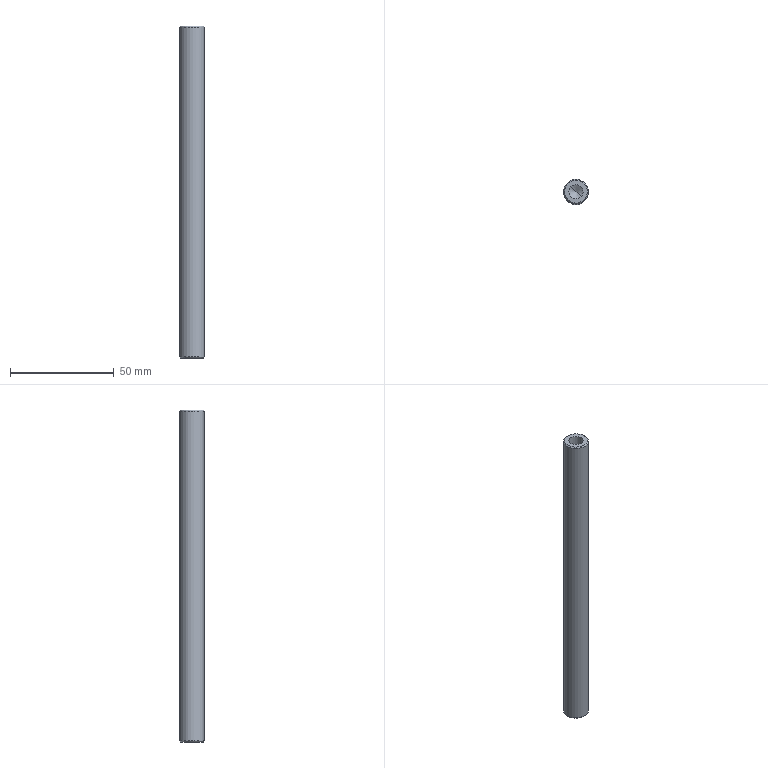Component | SolidWorks | TAR-02-081PaperRollAxis-1 | 1 solid | 12 faces | box 12 x 12 x 160 mm | volume 17018 mm3 | cone 6 | cylinder 4 | plane 2 | commonest cylinder face diameters 6.8 x2 12 x2
build123d program:
from build123d import *

# Parameters (mm, degrees)
SKETCH1_R             = 6
BOSS_EXTRUDE1_DEPTH   = 160
CHAMFER1_SIZE         = 0.5
M8_TAPPED_HOLE1_D     = 6.8
M8_TAPPED_HOLE1_DEPTH = 28.75
M8_TAPPED_HOLE1_TIP   = 2.043


with BuildPart() as part:
    # Sketch1 → Boss-Extrude1 (new body)
    with BuildSketch(Plane(origin=(0, 0, 0), x_dir=(0, 0, -1), z_dir=(1, 0, 0))):
        Circle(SKETCH1_R)
    extrude(amount=BOSS_EXTRUDE1_DEPTH)

    # Chamfer1
    chamfer1_edges = [part.edges().sort_by_distance(p)[0] for p in [
        (0, 0, 6),
        (160, 0, 6),
    ]]
    chamfer(chamfer1_edges, length=CHAMFER1_SIZE)

    # M8 Tapped Hole1
    with Locations(Plane(origin=(160, 0, 0), x_dir=(0, 0, 1), z_dir=(1, 0, 0))):
        with Locations((0, 0)):
            Hole(M8_TAPPED_HOLE1_D / 2, depth=M8_TAPPED_HOLE1_DEPTH)
            with Locations((0, 0, -(M8_TAPPED_HOLE1_DEPTH + M8_TAPPED_HOLE1_TIP / 2))):  # 118° drill point
                Cone(0, M8_TAPPED_HOLE1_D / 2, M8_TAPPED_HOLE1_TIP, mode=Mode.SUBTRACT)


solid = part.part

# Placed as in the assembly
solid = solid.moved(Location((-45.891, 68.788, -159.5), (0, -90, 0)))
STEP:
#1=COLOUR_RGB('',0.7922,0.8196,0.9333);
#2=FILL_AREA_STYLE_COLOUR('',#1);
#3=FILL_AREA_STYLE('',(#2));
#4=SURFACE_STYLE_FILL_AREA(#3);
#5=SURFACE_SIDE_STYLE('',(#4));
#6=SURFACE_STYLE_USAGE(.BOTH.,#5);
#7=PRESENTATION_STYLE_ASSIGNMENT((#6));
#8=CARTESIAN_POINT('',(-1.903,2.802,-1.112));
#9=VERTEX_POINT('',#8);
#10=CARTESIAN_POINT('',(-1.711,2.615,-1.112));
#11=VERTEX_POINT('',#10);
#12=CARTESIAN_POINT('',(-1.807,2.708,-1.112));
#13=DIRECTION('',(-0.,-0.,1.));
#14=DIRECTION('',(0.7165,-0.6976,0.));
#15=AXIS2_PLACEMENT_3D('',#12,#13,#14);
#16=CIRCLE('',#15,0.1339);
#17=EDGE_CURVE('',#9,#11,#16,.T.);
#18=ORIENTED_EDGE('',*,*,#17,.F.);
#19=CARTESIAN_POINT('',(-1.903,2.802,0.01969));
#20=VERTEX_POINT('',#19);
#21=CARTESIAN_POINT('',(-1.903,2.802,0.01969));
#22=DIRECTION('',(-0.,-0.,1.));
#23=VECTOR('',#22,39.37);
#24=LINE('',#21,#23);
#25=EDGE_CURVE('',#9,#20,#24,.T.);
#26=ORIENTED_EDGE('',*,*,#25,.T.);
#27=CARTESIAN_POINT('',(-1.711,2.615,0.01969));
#28=VERTEX_POINT('',#27);
#29=CARTESIAN_POINT('',(-1.807,2.708,0.01969));
#30=DIRECTION('',(-0.,-0.,1.));
#31=DIRECTION('',(0.7165,-0.6976,0.));
#32=AXIS2_PLACEMENT_3D('',#29,#30,#31);
#33=CIRCLE('',#32,0.1339);
#34=EDGE_CURVE('',#20,#28,#33,.T.);
#35=ORIENTED_EDGE('',*,*,#34,.T.);
#36=CARTESIAN_POINT('',(-1.711,2.615,0.01969));
#37=DIRECTION('',(-0.,-0.,1.));
#38=VECTOR('',#37,39.37);
#39=LINE('',#36,#38);
#40=EDGE_CURVE('',#11,#28,#39,.T.);
#41=ORIENTED_EDGE('',*,*,#40,.F.);
#42=EDGE_LOOP('',(#18,#26,#35,#41));
#43=FACE_OUTER_BOUND('',#42,.T.);
#44=CARTESIAN_POINT('',(-1.807,2.708,0.01969));
#45=DIRECTION('',(-0.,-0.,1.));
#46=DIRECTION('',(0.7165,-0.6976,0.));
#47=AXIS2_PLACEMENT_3D('',#44,#45,#46);
#48=CYLINDRICAL_SURFACE('',#47,0.1339);
#49=ADVANCED_FACE('',(#43),#48,.F.);
#50=CARTESIAN_POINT('',(-1.807,2.708,-1.193));
#51=VERTEX_POINT('',#50);
#52=CARTESIAN_POINT('',(-1.711,2.615,-1.112));
#53=DIRECTION('',(0.6142,-0.598,0.515));
#54=VECTOR('',#53,39.37);
#55=LINE('',#52,#54);
#56=EDGE_CURVE('',#51,#11,#55,.T.);
#57=ORIENTED_EDGE('',*,*,#56,.F.);
#58=CARTESIAN_POINT('',(-1.903,2.802,-1.112));
#59=DIRECTION('',(-0.6142,0.598,0.515));
#60=VECTOR('',#59,39.37);
#61=LINE('',#58,#60);
#62=EDGE_CURVE('',#51,#9,#61,.T.);
#63=ORIENTED_EDGE('',*,*,#62,.T.);
#64=ORIENTED_EDGE('',*,*,#17,.T.);
#65=EDGE_LOOP('',(#57,#63,#64));
#66=FACE_OUTER_BOUND('',#65,.T.);
#67=CARTESIAN_POINT('',(-1.807,2.708,-1.112));
#68=DIRECTION('',(-0.,-0.,1.));
#69=DIRECTION('',(0.7165,-0.6976,0.));
#70=AXIS2_PLACEMENT_3D('',#67,#68,#69);
#71=CONICAL_SURFACE('',#70,0.1339,1.03);
#72=ADVANCED_FACE('',(#66),#71,.F.);
#73=CARTESIAN_POINT('',(-1.652,2.557,0.01969));
#74=VERTEX_POINT('',#73);
#75=CARTESIAN_POINT('',(-1.962,2.859,0.01969));
#76=VERTEX_POINT('',#75);
#77=CARTESIAN_POINT('',(-1.807,2.708,0.01969));
#78=DIRECTION('',(-0.,-0.,1.));
#79=DIRECTION('',(0.7165,-0.6976,0.));
#80=AXIS2_PLACEMENT_3D('',#77,#78,#79);
#81=CIRCLE('',#80,0.2165);
#82=EDGE_CURVE('',#74,#76,#81,.T.);
#83=ORIENTED_EDGE('',*,*,#82,.F.);
#84=CARTESIAN_POINT('',(-1.637,2.543,-0.));
#85=VERTEX_POINT('',#84);
#86=CARTESIAN_POINT('',(-1.652,2.557,0.01969));
#87=DIRECTION('',(0.5066,-0.4933,-0.7071));
#88=VECTOR('',#87,39.37);
#89=LINE('',#86,#88);
#90=EDGE_CURVE('',#74,#85,#89,.T.);
#91=ORIENTED_EDGE('',*,*,#90,.T.);
#92=CARTESIAN_POINT('',(-1.976,2.873,-0.));
#93=VERTEX_POINT('',#92);
#94=CARTESIAN_POINT('',(-1.807,2.708,-0.));
#95=DIRECTION('',(0.,0.,-1.));
#96=DIRECTION('',(0.7165,-0.6976,0.));
#97=AXIS2_PLACEMENT_3D('',#94,#95,#96);
#98=CIRCLE('',#97,0.2362);
#99=EDGE_CURVE('',#93,#85,#98,.T.);
#100=ORIENTED_EDGE('',*,*,#99,.F.);
#101=CARTESIAN_POINT('',(-1.962,2.859,0.01969));
#102=DIRECTION('',(-0.5066,0.4933,-0.7071));
#103=VECTOR('',#102,39.37);
#104=LINE('',#101,#103);
#105=EDGE_CURVE('',#76,#93,#104,.T.);
#106=ORIENTED_EDGE('',*,*,#105,.F.);
#107=EDGE_LOOP('',(#83,#91,#100,#106));
#108=FACE_OUTER_BOUND('',#107,.T.);
#109=CARTESIAN_POINT('',(-1.807,2.708,0.01969));
#110=DIRECTION('',(0.,0.,-1.));
#111=DIRECTION('',(-0.7165,0.6976,-0.));
#112=AXIS2_PLACEMENT_3D('',#109,#110,#111);
#113=CONICAL_SURFACE('',#112,0.2165,0.7854);
#114=ADVANCED_FACE('',(#108),#113,.T.);
#115=CARTESIAN_POINT('',(-1.962,2.859,-6.28));
#116=VERTEX_POINT('',#115);
#117=CARTESIAN_POINT('',(-1.652,2.557,-6.28));
#118=VERTEX_POINT('',#117);
#119=CARTESIAN_POINT('',(-1.807,2.708,-6.28));
#120=DIRECTION('',(0.,0.,-1.));
#121=DIRECTION('',(0.7165,-0.6976,0.));
#122=AXIS2_PLACEMENT_3D('',#119,#120,#121);
#123=CIRCLE('',#122,0.2165);
#124=EDGE_CURVE('',#116,#118,#123,.T.);
#125=ORIENTED_EDGE('',*,*,#124,.F.);
#126=CARTESIAN_POINT('',(-1.976,2.873,-6.26));
#127=VERTEX_POINT('',#126);
#128=CARTESIAN_POINT('',(-1.976,2.873,-6.26));
#129=DIRECTION('',(-0.5066,0.4933,0.7071));
#130=VECTOR('',#129,39.37);
#131=LINE('',#128,#130);
#132=EDGE_CURVE('',#116,#127,#131,.T.);
#133=ORIENTED_EDGE('',*,*,#132,.T.);
#134=CARTESIAN_POINT('',(-1.637,2.543,-6.26));
#135=VERTEX_POINT('',#134);
#136=CARTESIAN_POINT('',(-1.807,2.708,-6.26));
#137=DIRECTION('',(-0.,-0.,1.));
#138=DIRECTION('',(0.7165,-0.6976,0.));
#139=AXIS2_PLACEMENT_3D('',#136,#137,#138);
#140=CIRCLE('',#139,0.2362);
#141=EDGE_CURVE('',#135,#127,#140,.T.);
#142=ORIENTED_EDGE('',*,*,#141,.F.);
#143=CARTESIAN_POINT('',(-1.637,2.543,-6.26));
#144=DIRECTION('',(0.5066,-0.4933,0.7071));
#145=VECTOR('',#144,39.37);
#146=LINE('',#143,#145);
#147=EDGE_CURVE('',#118,#135,#146,.T.);
#148=ORIENTED_EDGE('',*,*,#147,.F.);
#149=EDGE_LOOP('',(#125,#133,#142,#148));
#150=FACE_OUTER_BOUND('',#149,.T.);
#151=CARTESIAN_POINT('',(-1.807,2.708,-6.26));
#152=DIRECTION('',(-0.,-0.,1.));
#153=DIRECTION('',(0.7165,-0.6976,0.));
#154=AXIS2_PLACEMENT_3D('',#151,#152,#153);
#155=CONICAL_SURFACE('',#154,0.2362,0.7854);
#156=ADVANCED_FACE('',(#150),#155,.T.);
#157=ORIENTED_EDGE('',*,*,#99,.T.);
#158=CARTESIAN_POINT('',(-1.637,2.543,0.01969));
#159=DIRECTION('',(0.,0.,-1.));
#160=VECTOR('',#159,39.37);
#161=LINE('',#158,#160);
#162=EDGE_CURVE('',#85,#135,#161,.T.);
#163=ORIENTED_EDGE('',*,*,#162,.T.);
#164=ORIENTED_EDGE('',*,*,#141,.T.);
#165=CARTESIAN_POINT('',(-1.976,2.873,0.01969));
#166=DIRECTION('',(0.,0.,-1.));
#167=VECTOR('',#166,39.37);
#168=LINE('',#165,#167);
#169=EDGE_CURVE('',#93,#127,#168,.T.);
#170=ORIENTED_EDGE('',*,*,#169,.F.);
#171=EDGE_LOOP('',(#157,#163,#164,#170));
#172=FACE_OUTER_BOUND('',#171,.T.);
#173=CARTESIAN_POINT('',(-1.807,2.708,0.01969));
#174=DIRECTION('',(0.,0.,-1.));
#175=DIRECTION('',(-0.7165,0.6976,-0.));
#176=AXIS2_PLACEMENT_3D('',#173,#174,#175);
#177=CYLINDRICAL_SURFACE('',#176,0.2362);
#178=ADVANCED_FACE('',(#172),#177,.T.);
#179=ORIENTED_EDGE('',*,*,#162,.F.);
#180=CARTESIAN_POINT('',(-1.807,2.708,-0.));
#181=DIRECTION('',(0.,0.,-1.));
#182=DIRECTION('',(0.7165,-0.6976,0.));
#183=AXIS2_PLACEMENT_3D('',#180,#181,#182);
#184=CIRCLE('',#183,0.2362);
#185=EDGE_CURVE('',#85,#93,#184,.T.);
#186=ORIENTED_EDGE('',*,*,#185,.T.);
#187=ORIENTED_EDGE('',*,*,#169,.T.);
#188=CARTESIAN_POINT('',(-1.807,2.708,-6.26));
#189=DIRECTION('',(-0.,-0.,1.));
#190=DIRECTION('',(0.7165,-0.6976,0.));
#191=AXIS2_PLACEMENT_3D('',#188,#189,#190);
#192=CIRCLE('',#191,0.2362);
#193=EDGE_CURVE('',#127,#135,#192,.T.);
#194=ORIENTED_EDGE('',*,*,#193,.T.);
#195=EDGE_LOOP('',(#179,#186,#187,#194));
#196=FACE_OUTER_BOUND('',#195,.T.);
#197=CARTESIAN_POINT('',(-1.807,2.708,0.01969));
#198=DIRECTION('',(0.,0.,-1.));
#199=DIRECTION('',(-0.7165,0.6976,-0.));
#200=AXIS2_PLACEMENT_3D('',#197,#198,#199);
#201=CYLINDRICAL_SURFACE('',#200,0.2362);
#202=ADVANCED_FACE('',(#196),#201,.T.);
#203=CARTESIAN_POINT('',(-1.807,2.708,0.01969));
#204=DIRECTION('',(-0.,-0.,1.));
#205=DIRECTION('',(0.7165,-0.6976,0.));
#206=AXIS2_PLACEMENT_3D('',#203,#204,#205);
#207=CIRCLE('',#206,0.1339);
#208=EDGE_CURVE('',#28,#20,#207,.T.);
#209=ORIENTED_EDGE('',*,*,#208,.F.);
#210=ORIENTED_EDGE('',*,*,#34,.F.);
#211=EDGE_LOOP('',(#209,#210));
#212=FACE_BOUND('',#211,.T.);
#213=CARTESIAN_POINT('',(-1.807,2.708,0.01969));
#214=DIRECTION('',(-0.,-0.,1.));
#215=DIRECTION('',(0.7165,-0.6976,0.));
#216=AXIS2_PLACEMENT_3D('',#213,#214,#215);
#217=CIRCLE('',#216,0.2165);
#218=EDGE_CURVE('',#76,#74,#217,.T.);
#219=ORIENTED_EDGE('',*,*,#218,.T.);
#220=ORIENTED_EDGE('',*,*,#82,.T.);
#221=EDGE_LOOP('',(#219,#220));
#222=FACE_OUTER_BOUND('',#221,.T.);
#223=CARTESIAN_POINT('',(-1.807,2.708,0.01969));
#224=DIRECTION('',(-0.,-0.,1.));
#225=DIRECTION('',(0.7165,-0.6976,0.));
#226=AXIS2_PLACEMENT_3D('',#223,#224,#225);
#227=PLANE('',#226);
#228=ADVANCED_FACE('',(#212,#222),#227,.T.);
#229=CARTESIAN_POINT('',(-1.807,2.708,-6.28));
#230=DIRECTION('',(0.,0.,-1.));
#231=DIRECTION('',(0.7165,-0.6976,0.));
#232=AXIS2_PLACEMENT_3D('',#229,#230,#231);
#233=CIRCLE('',#232,0.2165);
#234=EDGE_CURVE('',#118,#116,#233,.T.);
#235=ORIENTED_EDGE('',*,*,#234,.T.);
#236=ORIENTED_EDGE('',*,*,#124,.T.);
#237=EDGE_LOOP('',(#235,#236));
#238=FACE_OUTER_BOUND('',#237,.T.);
#239=CARTESIAN_POINT('',(-1.807,2.708,-6.28));
#240=DIRECTION('',(-0.,-0.,1.));
#241=DIRECTION('',(0.7165,-0.6976,0.));
#242=AXIS2_PLACEMENT_3D('',#239,#240,#241);
#243=PLANE('',#242);
#244=ADVANCED_FACE('',(#238),#243,.F.);
#245=ORIENTED_EDGE('',*,*,#132,.F.);
#246=ORIENTED_EDGE('',*,*,#234,.F.);
#247=ORIENTED_EDGE('',*,*,#147,.T.);
#248=ORIENTED_EDGE('',*,*,#193,.F.);
#249=EDGE_LOOP('',(#245,#246,#247,#248));
#250=FACE_OUTER_BOUND('',#249,.T.);
#251=CARTESIAN_POINT('',(-1.807,2.708,-6.26));
#252=DIRECTION('',(-0.,-0.,1.));
#253=DIRECTION('',(0.7165,-0.6976,0.));
#254=AXIS2_PLACEMENT_3D('',#251,#252,#253);
#255=CONICAL_SURFACE('',#254,0.2362,0.7854);
#256=ADVANCED_FACE('',(#250),#255,.T.);
#257=ORIENTED_EDGE('',*,*,#90,.F.);
#258=ORIENTED_EDGE('',*,*,#218,.F.);
#259=ORIENTED_EDGE('',*,*,#105,.T.);
#260=ORIENTED_EDGE('',*,*,#185,.F.);
#261=EDGE_LOOP('',(#257,#258,#259,#260));
#262=FACE_OUTER_BOUND('',#261,.T.);
#263=CARTESIAN_POINT('',(-1.807,2.708,0.01969));
#264=DIRECTION('',(0.,0.,-1.));
#265=DIRECTION('',(-0.7165,0.6976,-0.));
#266=AXIS2_PLACEMENT_3D('',#263,#264,#265);
#267=CONICAL_SURFACE('',#266,0.2165,0.7854);
#268=ADVANCED_FACE('',(#262),#267,.T.);
#269=ORIENTED_EDGE('',*,*,#62,.F.);
#270=ORIENTED_EDGE('',*,*,#56,.T.);
#271=CARTESIAN_POINT('',(-1.807,2.708,-1.112));
#272=DIRECTION('',(-0.,-0.,1.));
#273=DIRECTION('',(0.7165,-0.6976,0.));
#274=AXIS2_PLACEMENT_3D('',#271,#272,#273);
#275=CIRCLE('',#274,0.1339);
#276=EDGE_CURVE('',#11,#9,#275,.T.);
#277=ORIENTED_EDGE('',*,*,#276,.T.);
#278=EDGE_LOOP('',(#269,#270,#277));
#279=FACE_OUTER_BOUND('',#278,.T.);
#280=CARTESIAN_POINT('',(-1.807,2.708,-1.112));
#281=DIRECTION('',(-0.,-0.,1.));
#282=DIRECTION('',(0.7165,-0.6976,0.));
#283=AXIS2_PLACEMENT_3D('',#280,#281,#282);
#284=CONICAL_SURFACE('',#283,0.1339,1.03);
#285=ADVANCED_FACE('',(#279),#284,.F.);
#286=ORIENTED_EDGE('',*,*,#25,.F.);
#287=ORIENTED_EDGE('',*,*,#276,.F.);
#288=ORIENTED_EDGE('',*,*,#40,.T.);
#289=ORIENTED_EDGE('',*,*,#208,.T.);
#290=EDGE_LOOP('',(#286,#287,#288,#289));
#291=FACE_OUTER_BOUND('',#290,.T.);
#292=CARTESIAN_POINT('',(-1.807,2.708,0.01969));
#293=DIRECTION('',(-0.,-0.,1.));
#294=DIRECTION('',(0.7165,-0.6976,0.));
#295=AXIS2_PLACEMENT_3D('',#292,#293,#294);
#296=CYLINDRICAL_SURFACE('',#295,0.1339);
#297=ADVANCED_FACE('',(#291),#296,.F.);
#298=CLOSED_SHELL('',(#49,#72,#114,#156,#178,#202,#228,#244,#256,#268,#285,#297));
#299=MANIFOLD_SOLID_BREP('',#298);
#300=STYLED_ITEM('',(#7),#299);
#301=PRESENTATION_LAYER_ASSIGNMENT('','',(#300));
#302=CARTESIAN_POINT('',(0.,0.,0.));
#303=DIRECTION('',(0.,0.,1.));
#304=DIRECTION('',(1.,0.,0.));
#305=AXIS2_PLACEMENT_3D('',#302,#303,#304);
#306=(LENGTH_UNIT()NAMED_UNIT(*)SI_UNIT($,.METRE.));
#307=LENGTH_MEASURE_WITH_UNIT(LENGTH_MEASURE(0.0254),#306);
#308=DIMENSIONAL_EXPONENTS(1.,0.,0.,0.,0.,0.,0.);
#309=(CONVERSION_BASED_UNIT('',#307)LENGTH_UNIT()NAMED_UNIT(#308));
#310=UNCERTAINTY_MEASURE_WITH_UNIT(LENGTH_MEASURE(0.00001),#309,'','');
#311=(NAMED_UNIT(*)PLANE_ANGLE_UNIT()SI_UNIT($,.RADIAN.));
#312=(NAMED_UNIT(*)SI_UNIT($,.STERADIAN.)SOLID_ANGLE_UNIT());
#313=(GEOMETRIC_REPRESENTATION_CONTEXT(3)GLOBAL_UNCERTAINTY_ASSIGNED_CONTEXT((#310))GLOBAL_UNIT_ASSIGNED_CONTEXT((#309,#311,#312))REPRESENTATION_CONTEXT('',''));
#314=ADVANCED_BREP_SHAPE_REPRESENTATION('',(#299,#305),#313);
#315=(LENGTH_UNIT()NAMED_UNIT(*)SI_UNIT($,.METRE.));
#316=LENGTH_MEASURE_WITH_UNIT(LENGTH_MEASURE(0.0254),#315);
#317=DIMENSIONAL_EXPONENTS(1.,0.,0.,0.,0.,0.,0.);
#318=(CONVERSION_BASED_UNIT('',#316)LENGTH_UNIT()NAMED_UNIT(#317));
#319=UNCERTAINTY_MEASURE_WITH_UNIT(LENGTH_MEASURE(0.00001),#318,'','');
#320=(NAMED_UNIT(*)PLANE_ANGLE_UNIT()SI_UNIT($,.RADIAN.));
#321=(NAMED_UNIT(*)SI_UNIT($,.STERADIAN.)SOLID_ANGLE_UNIT());
#322=(GEOMETRIC_REPRESENTATION_CONTEXT(3)GLOBAL_UNCERTAINTY_ASSIGNED_CONTEXT((#319))GLOBAL_UNIT_ASSIGNED_CONTEXT((#318,#320,#321))REPRESENTATION_CONTEXT('',''));
#323=MECHANICAL_DESIGN_GEOMETRIC_PRESENTATION_REPRESENTATION('',(#300),#322);